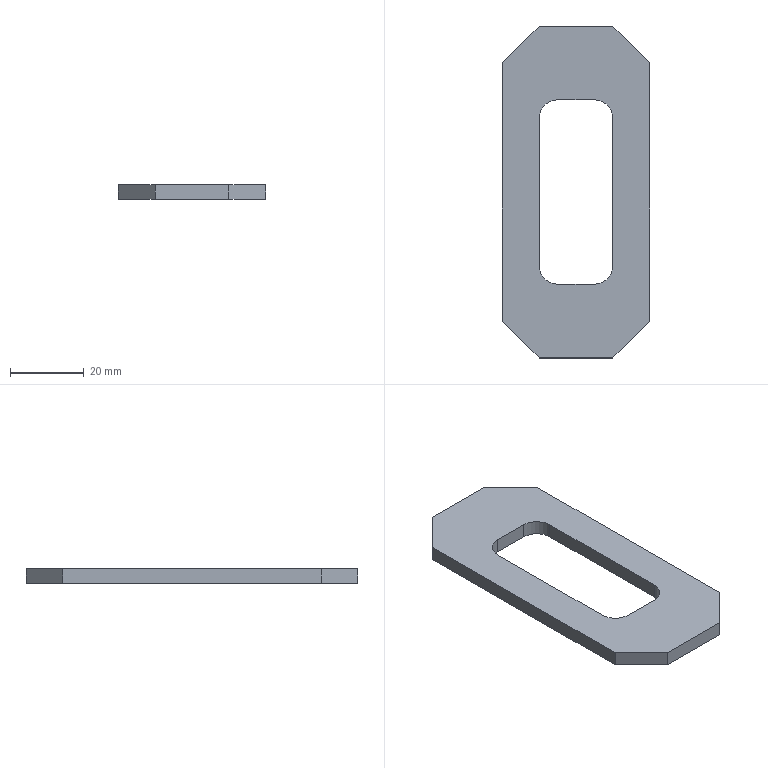Component | SolidWorks | THK-A1029RectangularTubeInnerSealingPlate-2 | 1 solid | 18 faces | box 40 x 90 x 4 mm | volume 9686 mm3 | plane 14 | cylinder 4 | commonest cylinder face diameters 10 x4 | material Q235A
build123d program:
from build123d import *

# Parameters (mm, degrees)
SKETCH1_W           = 40
SKETCH1_H           = 90
BOSS_EXTRUDE1_DEPTH = 2
CUT_EXTRUDE1_DEPTH  = 50.406
CHAMFER1_SIZE       = 10


with BuildPart() as part:
    # Sketch1 → Boss-Extrude1 (new, symmetric)
    with BuildSketch(Plane.XY):
        Rectangle(SKETCH1_W, SKETCH1_H)
    extrude(amount=BOSS_EXTRUDE1_DEPTH, both=True)

    # Sketch2 → Cut-Extrude1 (cut, through all)
    with BuildSketch(Plane.XY.offset(2)):
        with BuildLine():
            Line((-5, -25), (5, -25))
            ThreePointArc((5, -25), (8.536, -23.536), (10, -20))
            Line((10, -20), (10, 20))
            ThreePointArc((10, 20), (8.536, 23.536), (5, 25))
            Line((5, 25), (-5, 25))
            ThreePointArc((-5, 25), (-8.536, 23.536), (-10, 20))
            Line((-10, 20), (-10, -20))
            ThreePointArc((-10, -20), (-8.536, -23.536), (-5, -25))
        make_face()
    extrude(amount=-CUT_EXTRUDE1_DEPTH, mode=Mode.SUBTRACT)

    # Chamfer1
    chamfer1_edges = [part.edges().sort_by_distance(p)[0] for p in [
        (20, -45, 0),
        (-20, -45, 0),
        (-20, 45, 0),
        (20, 45, 0),
    ]]
    chamfer(chamfer1_edges, length=CHAMFER1_SIZE)


solid = part.part

# Placed as in the assembly
solid = solid.moved(Location((-155, -105, -293), (0, 0, 0)))
STEP:
#1=CARTESIAN_POINT('',(-5.315,-5.512,-11.457));
#2=VERTEX_POINT('',#1);
#3=CARTESIAN_POINT('',(-5.315,-2.756,-11.457));
#4=VERTEX_POINT('',#3);
#5=CARTESIAN_POINT('',(-5.315,-5.906,-11.457));
#6=DIRECTION('',(0.,1.,0.));
#7=VECTOR('',#6,39.37);
#8=LINE('',#5,#7);
#9=EDGE_CURVE('',#2,#4,#8,.T.);
#10=ORIENTED_EDGE('',*,*,#9,.F.);
#11=CARTESIAN_POINT('',(-5.315,-5.512,-11.614));
#12=VERTEX_POINT('',#11);
#13=CARTESIAN_POINT('',(-5.315,-5.512,-11.457));
#14=DIRECTION('',(0.,0.,-1.));
#15=VECTOR('',#14,39.37);
#16=LINE('',#13,#15);
#17=EDGE_CURVE('',#2,#12,#16,.T.);
#18=ORIENTED_EDGE('',*,*,#17,.T.);
#19=CARTESIAN_POINT('',(-5.315,-2.756,-11.614));
#20=VERTEX_POINT('',#19);
#21=CARTESIAN_POINT('',(-5.315,-5.906,-11.614));
#22=DIRECTION('',(0.,1.,0.));
#23=VECTOR('',#22,39.37);
#24=LINE('',#21,#23);
#25=EDGE_CURVE('',#12,#20,#24,.T.);
#26=ORIENTED_EDGE('',*,*,#25,.T.);
#27=CARTESIAN_POINT('',(-5.315,-2.756,-11.457));
#28=DIRECTION('',(0.,0.,1.));
#29=VECTOR('',#28,39.37);
#30=LINE('',#27,#29);
#31=EDGE_CURVE('',#20,#4,#30,.T.);
#32=ORIENTED_EDGE('',*,*,#31,.T.);
#33=EDGE_LOOP('',(#10,#18,#26,#32));
#34=FACE_OUTER_BOUND('',#33,.T.);
#35=CARTESIAN_POINT('',(-5.315,-5.906,-11.457));
#36=DIRECTION('',(-1.,0.,0.));
#37=DIRECTION('',(0.,0.,1.));
#38=AXIS2_PLACEMENT_3D('',#35,#36,#37);
#39=PLANE('',#38);
#40=ADVANCED_FACE('',(#34),#39,.F.);
#41=CARTESIAN_POINT('',(-5.709,-2.362,-11.614));
#42=VERTEX_POINT('',#41);
#43=CARTESIAN_POINT('',(-6.496,-2.362,-11.614));
#44=VERTEX_POINT('',#43);
#45=CARTESIAN_POINT('',(-6.89,-2.362,-11.614));
#46=DIRECTION('',(-1.,0.,0.));
#47=VECTOR('',#46,39.37);
#48=LINE('',#45,#47);
#49=EDGE_CURVE('',#42,#44,#48,.T.);
#50=ORIENTED_EDGE('',*,*,#49,.T.);
#51=CARTESIAN_POINT('',(-6.496,-2.362,-11.457));
#52=VERTEX_POINT('',#51);
#53=CARTESIAN_POINT('',(-6.496,-2.362,-11.457));
#54=DIRECTION('',(0.,0.,1.));
#55=VECTOR('',#54,39.37);
#56=LINE('',#53,#55);
#57=EDGE_CURVE('',#44,#52,#56,.T.);
#58=ORIENTED_EDGE('',*,*,#57,.T.);
#59=CARTESIAN_POINT('',(-5.709,-2.362,-11.457));
#60=VERTEX_POINT('',#59);
#61=CARTESIAN_POINT('',(-6.89,-2.362,-11.457));
#62=DIRECTION('',(-1.,0.,0.));
#63=VECTOR('',#62,39.37);
#64=LINE('',#61,#63);
#65=EDGE_CURVE('',#60,#52,#64,.T.);
#66=ORIENTED_EDGE('',*,*,#65,.F.);
#67=CARTESIAN_POINT('',(-5.709,-2.362,-11.457));
#68=DIRECTION('',(0.,0.,-1.));
#69=VECTOR('',#68,39.37);
#70=LINE('',#67,#69);
#71=EDGE_CURVE('',#60,#42,#70,.T.);
#72=ORIENTED_EDGE('',*,*,#71,.T.);
#73=EDGE_LOOP('',(#50,#58,#66,#72));
#74=FACE_OUTER_BOUND('',#73,.T.);
#75=CARTESIAN_POINT('',(-6.89,-2.362,-11.457));
#76=DIRECTION('',(0.,-1.,0.));
#77=DIRECTION('',(0.,0.,-1.));
#78=AXIS2_PLACEMENT_3D('',#75,#76,#77);
#79=PLANE('',#78);
#80=ADVANCED_FACE('',(#74),#79,.F.);
#81=CARTESIAN_POINT('',(-6.89,-2.756,-11.614));
#82=VERTEX_POINT('',#81);
#83=CARTESIAN_POINT('',(-6.89,-5.512,-11.614));
#84=VERTEX_POINT('',#83);
#85=CARTESIAN_POINT('',(-6.89,-5.906,-11.614));
#86=DIRECTION('',(0.,-1.,0.));
#87=VECTOR('',#86,39.37);
#88=LINE('',#85,#87);
#89=EDGE_CURVE('',#82,#84,#88,.T.);
#90=ORIENTED_EDGE('',*,*,#89,.T.);
#91=CARTESIAN_POINT('',(-6.89,-5.512,-11.457));
#92=VERTEX_POINT('',#91);
#93=CARTESIAN_POINT('',(-6.89,-5.512,-11.457));
#94=DIRECTION('',(0.,0.,1.));
#95=VECTOR('',#94,39.37);
#96=LINE('',#93,#95);
#97=EDGE_CURVE('',#84,#92,#96,.T.);
#98=ORIENTED_EDGE('',*,*,#97,.T.);
#99=CARTESIAN_POINT('',(-6.89,-2.756,-11.457));
#100=VERTEX_POINT('',#99);
#101=CARTESIAN_POINT('',(-6.89,-5.906,-11.457));
#102=DIRECTION('',(0.,-1.,0.));
#103=VECTOR('',#102,39.37);
#104=LINE('',#101,#103);
#105=EDGE_CURVE('',#100,#92,#104,.T.);
#106=ORIENTED_EDGE('',*,*,#105,.F.);
#107=CARTESIAN_POINT('',(-6.89,-2.756,-11.457));
#108=DIRECTION('',(0.,0.,-1.));
#109=VECTOR('',#108,39.37);
#110=LINE('',#107,#109);
#111=EDGE_CURVE('',#100,#82,#110,.T.);
#112=ORIENTED_EDGE('',*,*,#111,.T.);
#113=EDGE_LOOP('',(#90,#98,#106,#112));
#114=FACE_OUTER_BOUND('',#113,.T.);
#115=CARTESIAN_POINT('',(-6.89,-5.906,-11.457));
#116=DIRECTION('',(1.,0.,0.));
#117=DIRECTION('',(0.,0.,-1.));
#118=AXIS2_PLACEMENT_3D('',#115,#116,#117);
#119=PLANE('',#118);
#120=ADVANCED_FACE('',(#114),#119,.F.);
#121=CARTESIAN_POINT('',(-6.496,-5.906,-11.614));
#122=VERTEX_POINT('',#121);
#123=CARTESIAN_POINT('',(-5.709,-5.906,-11.614));
#124=VERTEX_POINT('',#123);
#125=CARTESIAN_POINT('',(-6.89,-5.906,-11.614));
#126=DIRECTION('',(1.,0.,0.));
#127=VECTOR('',#126,39.37);
#128=LINE('',#125,#127);
#129=EDGE_CURVE('',#122,#124,#128,.T.);
#130=ORIENTED_EDGE('',*,*,#129,.T.);
#131=CARTESIAN_POINT('',(-5.709,-5.906,-11.457));
#132=VERTEX_POINT('',#131);
#133=CARTESIAN_POINT('',(-5.709,-5.906,-11.457));
#134=DIRECTION('',(0.,0.,1.));
#135=VECTOR('',#134,39.37);
#136=LINE('',#133,#135);
#137=EDGE_CURVE('',#124,#132,#136,.T.);
#138=ORIENTED_EDGE('',*,*,#137,.T.);
#139=CARTESIAN_POINT('',(-6.496,-5.906,-11.457));
#140=VERTEX_POINT('',#139);
#141=CARTESIAN_POINT('',(-6.89,-5.906,-11.457));
#142=DIRECTION('',(1.,0.,0.));
#143=VECTOR('',#142,39.37);
#144=LINE('',#141,#143);
#145=EDGE_CURVE('',#140,#132,#144,.T.);
#146=ORIENTED_EDGE('',*,*,#145,.F.);
#147=CARTESIAN_POINT('',(-6.496,-5.906,-11.457));
#148=DIRECTION('',(0.,0.,-1.));
#149=VECTOR('',#148,39.37);
#150=LINE('',#147,#149);
#151=EDGE_CURVE('',#140,#122,#150,.T.);
#152=ORIENTED_EDGE('',*,*,#151,.T.);
#153=EDGE_LOOP('',(#130,#138,#146,#152));
#154=FACE_OUTER_BOUND('',#153,.T.);
#155=CARTESIAN_POINT('',(-6.89,-5.906,-11.457));
#156=DIRECTION('',(0.,1.,0.));
#157=DIRECTION('',(0.,0.,1.));
#158=AXIS2_PLACEMENT_3D('',#155,#156,#157);
#159=PLANE('',#158);
#160=ADVANCED_FACE('',(#154),#159,.F.);
#161=CARTESIAN_POINT('',(-6.299,-5.118,-11.457));
#162=VERTEX_POINT('',#161);
#163=CARTESIAN_POINT('',(-5.906,-5.118,-11.457));
#164=VERTEX_POINT('',#163);
#165=CARTESIAN_POINT('',(-6.299,-5.118,-11.457));
#166=DIRECTION('',(1.,0.,0.));
#167=VECTOR('',#166,39.37);
#168=LINE('',#165,#167);
#169=EDGE_CURVE('',#162,#164,#168,.T.);
#170=ORIENTED_EDGE('',*,*,#169,.F.);
#171=CARTESIAN_POINT('',(-6.496,-4.921,-11.457));
#172=VERTEX_POINT('',#171);
#173=CARTESIAN_POINT('',(-6.299,-4.921,-11.457));
#174=DIRECTION('',(0.,0.,1.));
#175=DIRECTION('',(1.,0.,0.));
#176=AXIS2_PLACEMENT_3D('',#173,#174,#175);
#177=CIRCLE('',#176,0.1969);
#178=EDGE_CURVE('',#172,#162,#177,.T.);
#179=ORIENTED_EDGE('',*,*,#178,.F.);
#180=CARTESIAN_POINT('',(-6.496,-3.346,-11.457));
#181=VERTEX_POINT('',#180);
#182=CARTESIAN_POINT('',(-6.496,-4.921,-11.457));
#183=DIRECTION('',(0.,-1.,0.));
#184=VECTOR('',#183,39.37);
#185=LINE('',#182,#184);
#186=EDGE_CURVE('',#181,#172,#185,.T.);
#187=ORIENTED_EDGE('',*,*,#186,.F.);
#188=CARTESIAN_POINT('',(-6.299,-3.15,-11.457));
#189=VERTEX_POINT('',#188);
#190=CARTESIAN_POINT('',(-6.299,-3.346,-11.457));
#191=DIRECTION('',(0.,0.,1.));
#192=DIRECTION('',(-1.,0.,0.));
#193=AXIS2_PLACEMENT_3D('',#190,#191,#192);
#194=CIRCLE('',#193,0.1969);
#195=EDGE_CURVE('',#189,#181,#194,.T.);
#196=ORIENTED_EDGE('',*,*,#195,.F.);
#197=CARTESIAN_POINT('',(-5.906,-3.15,-11.457));
#198=VERTEX_POINT('',#197);
#199=CARTESIAN_POINT('',(-6.299,-3.15,-11.457));
#200=DIRECTION('',(-1.,0.,0.));
#201=VECTOR('',#200,39.37);
#202=LINE('',#199,#201);
#203=EDGE_CURVE('',#198,#189,#202,.T.);
#204=ORIENTED_EDGE('',*,*,#203,.F.);
#205=CARTESIAN_POINT('',(-5.709,-3.346,-11.457));
#206=VERTEX_POINT('',#205);
#207=CARTESIAN_POINT('',(-5.906,-3.346,-11.457));
#208=DIRECTION('',(0.,0.,1.));
#209=DIRECTION('',(-1.,0.,0.));
#210=AXIS2_PLACEMENT_3D('',#207,#208,#209);
#211=CIRCLE('',#210,0.1969);
#212=EDGE_CURVE('',#206,#198,#211,.T.);
#213=ORIENTED_EDGE('',*,*,#212,.F.);
#214=CARTESIAN_POINT('',(-5.709,-4.921,-11.457));
#215=VERTEX_POINT('',#214);
#216=CARTESIAN_POINT('',(-5.709,-4.921,-11.457));
#217=DIRECTION('',(0.,1.,0.));
#218=VECTOR('',#217,39.37);
#219=LINE('',#216,#218);
#220=EDGE_CURVE('',#215,#206,#219,.T.);
#221=ORIENTED_EDGE('',*,*,#220,.F.);
#222=CARTESIAN_POINT('',(-5.906,-4.921,-11.457));
#223=DIRECTION('',(0.,0.,1.));
#224=DIRECTION('',(1.,0.,0.));
#225=AXIS2_PLACEMENT_3D('',#222,#223,#224);
#226=CIRCLE('',#225,0.1969);
#227=EDGE_CURVE('',#164,#215,#226,.T.);
#228=ORIENTED_EDGE('',*,*,#227,.F.);
#229=EDGE_LOOP('',(#170,#179,#187,#196,#204,#213,#221,#228));
#230=FACE_BOUND('',#229,.T.);
#231=ORIENTED_EDGE('',*,*,#145,.T.);
#232=CARTESIAN_POINT('',(-5.315,-5.512,-11.457));
#233=DIRECTION('',(0.7071,0.7071,0.));
#234=VECTOR('',#233,39.37);
#235=LINE('',#232,#234);
#236=EDGE_CURVE('',#132,#2,#235,.T.);
#237=ORIENTED_EDGE('',*,*,#236,.T.);
#238=ORIENTED_EDGE('',*,*,#9,.T.);
#239=CARTESIAN_POINT('',(-5.709,-2.362,-11.457));
#240=DIRECTION('',(-0.7071,0.7071,0.));
#241=VECTOR('',#240,39.37);
#242=LINE('',#239,#241);
#243=EDGE_CURVE('',#4,#60,#242,.T.);
#244=ORIENTED_EDGE('',*,*,#243,.T.);
#245=ORIENTED_EDGE('',*,*,#65,.T.);
#246=CARTESIAN_POINT('',(-6.89,-2.756,-11.457));
#247=DIRECTION('',(-0.7071,-0.7071,0.));
#248=VECTOR('',#247,39.37);
#249=LINE('',#246,#248);
#250=EDGE_CURVE('',#52,#100,#249,.T.);
#251=ORIENTED_EDGE('',*,*,#250,.T.);
#252=ORIENTED_EDGE('',*,*,#105,.T.);
#253=CARTESIAN_POINT('',(-6.496,-5.906,-11.457));
#254=DIRECTION('',(0.7071,-0.7071,0.));
#255=VECTOR('',#254,39.37);
#256=LINE('',#253,#255);
#257=EDGE_CURVE('',#92,#140,#256,.T.);
#258=ORIENTED_EDGE('',*,*,#257,.T.);
#259=EDGE_LOOP('',(#231,#237,#238,#244,#245,#251,#252,#258));
#260=FACE_OUTER_BOUND('',#259,.T.);
#261=CARTESIAN_POINT('',(-6.102,-4.134,-11.457));
#262=DIRECTION('',(0.,0.,-1.));
#263=DIRECTION('',(-1.,0.,0.));
#264=AXIS2_PLACEMENT_3D('',#261,#262,#263);
#265=PLANE('',#264);
#266=ADVANCED_FACE('',(#230,#260),#265,.F.);
#267=CARTESIAN_POINT('',(-6.496,-4.921,-11.614));
#268=VERTEX_POINT('',#267);
#269=CARTESIAN_POINT('',(-6.299,-5.118,-11.614));
#270=VERTEX_POINT('',#269);
#271=CARTESIAN_POINT('',(-6.299,-4.921,-11.614));
#272=DIRECTION('',(0.,0.,1.));
#273=DIRECTION('',(1.,0.,0.));
#274=AXIS2_PLACEMENT_3D('',#271,#272,#273);
#275=CIRCLE('',#274,0.1969);
#276=EDGE_CURVE('',#268,#270,#275,.T.);
#277=ORIENTED_EDGE('',*,*,#276,.T.);
#278=CARTESIAN_POINT('',(-5.906,-5.118,-11.614));
#279=VERTEX_POINT('',#278);
#280=CARTESIAN_POINT('',(-6.299,-5.118,-11.614));
#281=DIRECTION('',(1.,0.,0.));
#282=VECTOR('',#281,39.37);
#283=LINE('',#280,#282);
#284=EDGE_CURVE('',#270,#279,#283,.T.);
#285=ORIENTED_EDGE('',*,*,#284,.T.);
#286=CARTESIAN_POINT('',(-5.709,-4.921,-11.614));
#287=VERTEX_POINT('',#286);
#288=CARTESIAN_POINT('',(-5.906,-4.921,-11.614));
#289=DIRECTION('',(0.,0.,1.));
#290=DIRECTION('',(1.,0.,0.));
#291=AXIS2_PLACEMENT_3D('',#288,#289,#290);
#292=CIRCLE('',#291,0.1969);
#293=EDGE_CURVE('',#279,#287,#292,.T.);
#294=ORIENTED_EDGE('',*,*,#293,.T.);
#295=CARTESIAN_POINT('',(-5.709,-3.346,-11.614));
#296=VERTEX_POINT('',#295);
#297=CARTESIAN_POINT('',(-5.709,-4.921,-11.614));
#298=DIRECTION('',(0.,1.,0.));
#299=VECTOR('',#298,39.37);
#300=LINE('',#297,#299);
#301=EDGE_CURVE('',#287,#296,#300,.T.);
#302=ORIENTED_EDGE('',*,*,#301,.T.);
#303=CARTESIAN_POINT('',(-5.906,-3.15,-11.614));
#304=VERTEX_POINT('',#303);
#305=CARTESIAN_POINT('',(-5.906,-3.346,-11.614));
#306=DIRECTION('',(0.,0.,1.));
#307=DIRECTION('',(-1.,0.,0.));
#308=AXIS2_PLACEMENT_3D('',#305,#306,#307);
#309=CIRCLE('',#308,0.1969);
#310=EDGE_CURVE('',#296,#304,#309,.T.);
#311=ORIENTED_EDGE('',*,*,#310,.T.);
#312=CARTESIAN_POINT('',(-6.299,-3.15,-11.614));
#313=VERTEX_POINT('',#312);
#314=CARTESIAN_POINT('',(-6.299,-3.15,-11.614));
#315=DIRECTION('',(-1.,0.,0.));
#316=VECTOR('',#315,39.37);
#317=LINE('',#314,#316);
#318=EDGE_CURVE('',#304,#313,#317,.T.);
#319=ORIENTED_EDGE('',*,*,#318,.T.);
#320=CARTESIAN_POINT('',(-6.496,-3.346,-11.614));
#321=VERTEX_POINT('',#320);
#322=CARTESIAN_POINT('',(-6.299,-3.346,-11.614));
#323=DIRECTION('',(0.,0.,1.));
#324=DIRECTION('',(-1.,0.,0.));
#325=AXIS2_PLACEMENT_3D('',#322,#323,#324);
#326=CIRCLE('',#325,0.1969);
#327=EDGE_CURVE('',#313,#321,#326,.T.);
#328=ORIENTED_EDGE('',*,*,#327,.T.);
#329=CARTESIAN_POINT('',(-6.496,-4.921,-11.614));
#330=DIRECTION('',(0.,-1.,0.));
#331=VECTOR('',#330,39.37);
#332=LINE('',#329,#331);
#333=EDGE_CURVE('',#321,#268,#332,.T.);
#334=ORIENTED_EDGE('',*,*,#333,.T.);
#335=EDGE_LOOP('',(#277,#285,#294,#302,#311,#319,#328,#334));
#336=FACE_BOUND('',#335,.T.);
#337=ORIENTED_EDGE('',*,*,#25,.F.);
#338=CARTESIAN_POINT('',(-5.02,-5.217,-11.614));
#339=DIRECTION('',(-0.7071,-0.7071,0.));
#340=VECTOR('',#339,39.37);
#341=LINE('',#338,#340);
#342=EDGE_CURVE('',#12,#124,#341,.T.);
#343=ORIENTED_EDGE('',*,*,#342,.T.);
#344=ORIENTED_EDGE('',*,*,#129,.F.);
#345=CARTESIAN_POINT('',(-7.185,-5.217,-11.614));
#346=DIRECTION('',(-0.7071,0.7071,0.));
#347=VECTOR('',#346,39.37);
#348=LINE('',#345,#347);
#349=EDGE_CURVE('',#122,#84,#348,.T.);
#350=ORIENTED_EDGE('',*,*,#349,.T.);
#351=ORIENTED_EDGE('',*,*,#89,.F.);
#352=CARTESIAN_POINT('',(-7.185,-3.051,-11.614));
#353=DIRECTION('',(0.7071,0.7071,0.));
#354=VECTOR('',#353,39.37);
#355=LINE('',#352,#354);
#356=EDGE_CURVE('',#82,#44,#355,.T.);
#357=ORIENTED_EDGE('',*,*,#356,.T.);
#358=ORIENTED_EDGE('',*,*,#49,.F.);
#359=CARTESIAN_POINT('',(-5.02,-3.051,-11.614));
#360=DIRECTION('',(0.7071,-0.7071,0.));
#361=VECTOR('',#360,39.37);
#362=LINE('',#359,#361);
#363=EDGE_CURVE('',#42,#20,#362,.T.);
#364=ORIENTED_EDGE('',*,*,#363,.T.);
#365=EDGE_LOOP('',(#337,#343,#344,#350,#351,#357,#358,#364));
#366=FACE_OUTER_BOUND('',#365,.T.);
#367=CARTESIAN_POINT('',(-6.102,-4.134,-11.614));
#368=DIRECTION('',(0.,0.,-1.));
#369=DIRECTION('',(-1.,0.,0.));
#370=AXIS2_PLACEMENT_3D('',#367,#368,#369);
#371=PLANE('',#370);
#372=ADVANCED_FACE('',(#336,#366),#371,.T.);
#373=ORIENTED_EDGE('',*,*,#178,.T.);
#374=CARTESIAN_POINT('',(-6.299,-5.118,-11.614));
#375=DIRECTION('',(0.,0.,1.));
#376=VECTOR('',#375,39.37);
#377=LINE('',#374,#376);
#378=EDGE_CURVE('',#270,#162,#377,.T.);
#379=ORIENTED_EDGE('',*,*,#378,.F.);
#380=ORIENTED_EDGE('',*,*,#276,.F.);
#381=CARTESIAN_POINT('',(-6.496,-4.921,-11.614));
#382=DIRECTION('',(0.,0.,1.));
#383=VECTOR('',#382,39.37);
#384=LINE('',#381,#383);
#385=EDGE_CURVE('',#268,#172,#384,.T.);
#386=ORIENTED_EDGE('',*,*,#385,.T.);
#387=EDGE_LOOP('',(#373,#379,#380,#386));
#388=FACE_OUTER_BOUND('',#387,.T.);
#389=CARTESIAN_POINT('',(-6.299,-4.921,-11.614));
#390=DIRECTION('',(0.,0.,1.));
#391=DIRECTION('',(1.,0.,0.));
#392=AXIS2_PLACEMENT_3D('',#389,#390,#391);
#393=CYLINDRICAL_SURFACE('',#392,0.1969);
#394=ADVANCED_FACE('',(#388),#393,.F.);
#395=ORIENTED_EDGE('',*,*,#186,.T.);
#396=ORIENTED_EDGE('',*,*,#385,.F.);
#397=ORIENTED_EDGE('',*,*,#333,.F.);
#398=CARTESIAN_POINT('',(-6.496,-3.346,-11.614));
#399=DIRECTION('',(0.,0.,1.));
#400=VECTOR('',#399,39.37);
#401=LINE('',#398,#400);
#402=EDGE_CURVE('',#321,#181,#401,.T.);
#403=ORIENTED_EDGE('',*,*,#402,.T.);
#404=EDGE_LOOP('',(#395,#396,#397,#403));
#405=FACE_OUTER_BOUND('',#404,.T.);
#406=CARTESIAN_POINT('',(-6.496,-4.921,-11.614));
#407=DIRECTION('',(-1.,0.,0.));
#408=DIRECTION('',(0.,0.,1.));
#409=AXIS2_PLACEMENT_3D('',#406,#407,#408);
#410=PLANE('',#409);
#411=ADVANCED_FACE('',(#405),#410,.F.);
#412=ORIENTED_EDGE('',*,*,#195,.T.);
#413=ORIENTED_EDGE('',*,*,#402,.F.);
#414=ORIENTED_EDGE('',*,*,#327,.F.);
#415=CARTESIAN_POINT('',(-6.299,-3.15,-11.614));
#416=DIRECTION('',(0.,0.,1.));
#417=VECTOR('',#416,39.37);
#418=LINE('',#415,#417);
#419=EDGE_CURVE('',#313,#189,#418,.T.);
#420=ORIENTED_EDGE('',*,*,#419,.T.);
#421=EDGE_LOOP('',(#412,#413,#414,#420));
#422=FACE_OUTER_BOUND('',#421,.T.);
#423=CARTESIAN_POINT('',(-6.299,-3.346,-11.614));
#424=DIRECTION('',(0.,0.,1.));
#425=DIRECTION('',(1.,0.,0.));
#426=AXIS2_PLACEMENT_3D('',#423,#424,#425);
#427=CYLINDRICAL_SURFACE('',#426,0.1969);
#428=ADVANCED_FACE('',(#422),#427,.F.);
#429=ORIENTED_EDGE('',*,*,#203,.T.);
#430=ORIENTED_EDGE('',*,*,#419,.F.);
#431=ORIENTED_EDGE('',*,*,#318,.F.);
#432=CARTESIAN_POINT('',(-5.906,-3.15,-11.614));
#433=DIRECTION('',(0.,0.,1.));
#434=VECTOR('',#433,39.37);
#435=LINE('',#432,#434);
#436=EDGE_CURVE('',#304,#198,#435,.T.);
#437=ORIENTED_EDGE('',*,*,#436,.T.);
#438=EDGE_LOOP('',(#429,#430,#431,#437));
#439=FACE_OUTER_BOUND('',#438,.T.);
#440=CARTESIAN_POINT('',(-6.299,-3.15,-11.614));
#441=DIRECTION('',(0.,1.,0.));
#442=DIRECTION('',(0.,0.,1.));
#443=AXIS2_PLACEMENT_3D('',#440,#441,#442);
#444=PLANE('',#443);
#445=ADVANCED_FACE('',(#439),#444,.F.);
#446=ORIENTED_EDGE('',*,*,#212,.T.);
#447=ORIENTED_EDGE('',*,*,#436,.F.);
#448=ORIENTED_EDGE('',*,*,#310,.F.);
#449=CARTESIAN_POINT('',(-5.709,-3.346,-11.614));
#450=DIRECTION('',(0.,0.,1.));
#451=VECTOR('',#450,39.37);
#452=LINE('',#449,#451);
#453=EDGE_CURVE('',#296,#206,#452,.T.);
#454=ORIENTED_EDGE('',*,*,#453,.T.);
#455=EDGE_LOOP('',(#446,#447,#448,#454));
#456=FACE_OUTER_BOUND('',#455,.T.);
#457=CARTESIAN_POINT('',(-5.906,-3.346,-11.614));
#458=DIRECTION('',(0.,0.,1.));
#459=DIRECTION('',(1.,0.,0.));
#460=AXIS2_PLACEMENT_3D('',#457,#458,#459);
#461=CYLINDRICAL_SURFACE('',#460,0.1969);
#462=ADVANCED_FACE('',(#456),#461,.F.);
#463=ORIENTED_EDGE('',*,*,#220,.T.);
#464=ORIENTED_EDGE('',*,*,#453,.F.);
#465=ORIENTED_EDGE('',*,*,#301,.F.);
#466=CARTESIAN_POINT('',(-5.709,-4.921,-11.614));
#467=DIRECTION('',(0.,0.,1.));
#468=VECTOR('',#467,39.37);
#469=LINE('',#466,#468);
#470=EDGE_CURVE('',#287,#215,#469,.T.);
#471=ORIENTED_EDGE('',*,*,#470,.T.);
#472=EDGE_LOOP('',(#463,#464,#465,#471));
#473=FACE_OUTER_BOUND('',#472,.T.);
#474=CARTESIAN_POINT('',(-5.709,-4.921,-11.614));
#475=DIRECTION('',(1.,0.,0.));
#476=DIRECTION('',(0.,0.,-1.));
#477=AXIS2_PLACEMENT_3D('',#474,#475,#476);
#478=PLANE('',#477);
#479=ADVANCED_FACE('',(#473),#478,.F.);
#480=ORIENTED_EDGE('',*,*,#227,.T.);
#481=ORIENTED_EDGE('',*,*,#470,.F.);
#482=ORIENTED_EDGE('',*,*,#293,.F.);
#483=CARTESIAN_POINT('',(-5.906,-5.118,-11.614));
#484=DIRECTION('',(0.,0.,1.));
#485=VECTOR('',#484,39.37);
#486=LINE('',#483,#485);
#487=EDGE_CURVE('',#279,#164,#486,.T.);
#488=ORIENTED_EDGE('',*,*,#487,.T.);
#489=EDGE_LOOP('',(#480,#481,#482,#488));
#490=FACE_OUTER_BOUND('',#489,.T.);
#491=CARTESIAN_POINT('',(-5.906,-4.921,-11.614));
#492=DIRECTION('',(0.,0.,1.));
#493=DIRECTION('',(1.,0.,0.));
#494=AXIS2_PLACEMENT_3D('',#491,#492,#493);
#495=CYLINDRICAL_SURFACE('',#494,0.1969);
#496=ADVANCED_FACE('',(#490),#495,.F.);
#497=ORIENTED_EDGE('',*,*,#169,.T.);
#498=ORIENTED_EDGE('',*,*,#487,.F.);
#499=ORIENTED_EDGE('',*,*,#284,.F.);
#500=ORIENTED_EDGE('',*,*,#378,.T.);
#501=EDGE_LOOP('',(#497,#498,#499,#500));
#502=FACE_OUTER_BOUND('',#501,.T.);
#503=CARTESIAN_POINT('',(-6.299,-5.118,-11.614));
#504=DIRECTION('',(0.,-1.,0.));
#505=DIRECTION('',(0.,0.,-1.));
#506=AXIS2_PLACEMENT_3D('',#503,#504,#505);
#507=PLANE('',#506);
#508=ADVANCED_FACE('',(#502),#507,.F.);
#509=ORIENTED_EDGE('',*,*,#236,.F.);
#510=ORIENTED_EDGE('',*,*,#137,.F.);
#511=ORIENTED_EDGE('',*,*,#342,.F.);
#512=ORIENTED_EDGE('',*,*,#17,.F.);
#513=EDGE_LOOP('',(#509,#510,#511,#512));
#514=FACE_OUTER_BOUND('',#513,.T.);
#515=CARTESIAN_POINT('',(-5.315,-5.512,-11.457));
#516=DIRECTION('',(-0.7071,0.7071,0.));
#517=DIRECTION('',(0.,0.,-1.));
#518=AXIS2_PLACEMENT_3D('',#515,#516,#517);
#519=PLANE('',#518);
#520=ADVANCED_FACE('',(#514),#519,.F.);
#521=ORIENTED_EDGE('',*,*,#257,.F.);
#522=ORIENTED_EDGE('',*,*,#97,.F.);
#523=ORIENTED_EDGE('',*,*,#349,.F.);
#524=ORIENTED_EDGE('',*,*,#151,.F.);
#525=EDGE_LOOP('',(#521,#522,#523,#524));
#526=FACE_OUTER_BOUND('',#525,.T.);
#527=CARTESIAN_POINT('',(-6.496,-5.906,-11.457));
#528=DIRECTION('',(0.7071,0.7071,0.));
#529=DIRECTION('',(0.,0.,-1.));
#530=AXIS2_PLACEMENT_3D('',#527,#528,#529);
#531=PLANE('',#530);
#532=ADVANCED_FACE('',(#526),#531,.F.);
#533=ORIENTED_EDGE('',*,*,#250,.F.);
#534=ORIENTED_EDGE('',*,*,#57,.F.);
#535=ORIENTED_EDGE('',*,*,#356,.F.);
#536=ORIENTED_EDGE('',*,*,#111,.F.);
#537=EDGE_LOOP('',(#533,#534,#535,#536));
#538=FACE_OUTER_BOUND('',#537,.T.);
#539=CARTESIAN_POINT('',(-6.89,-2.756,-11.457));
#540=DIRECTION('',(0.7071,-0.7071,0.));
#541=DIRECTION('',(0.,0.,-1.));
#542=AXIS2_PLACEMENT_3D('',#539,#540,#541);
#543=PLANE('',#542);
#544=ADVANCED_FACE('',(#538),#543,.F.);
#545=ORIENTED_EDGE('',*,*,#243,.F.);
#546=ORIENTED_EDGE('',*,*,#31,.F.);
#547=ORIENTED_EDGE('',*,*,#363,.F.);
#548=ORIENTED_EDGE('',*,*,#71,.F.);
#549=EDGE_LOOP('',(#545,#546,#547,#548));
#550=FACE_OUTER_BOUND('',#549,.T.);
#551=CARTESIAN_POINT('',(-5.709,-2.362,-11.457));
#552=DIRECTION('',(-0.7071,-0.7071,0.));
#553=DIRECTION('',(0.,0.,-1.));
#554=AXIS2_PLACEMENT_3D('',#551,#552,#553);
#555=PLANE('',#554);
#556=ADVANCED_FACE('',(#550),#555,.F.);
#557=CLOSED_SHELL('',(#40,#80,#120,#160,#266,#372,#394,#411,#428,#445,#462,#479,#496,#508,#520,#532,#544,#556));
#558=MANIFOLD_SOLID_BREP('',#557);
#559=CARTESIAN_POINT('',(0.,0.,0.));
#560=DIRECTION('',(0.,0.,1.));
#561=DIRECTION('',(1.,0.,0.));
#562=AXIS2_PLACEMENT_3D('',#559,#560,#561);
#563=(LENGTH_UNIT()NAMED_UNIT(*)SI_UNIT($,.METRE.));
#564=LENGTH_MEASURE_WITH_UNIT(LENGTH_MEASURE(0.0254),#563);
#565=DIMENSIONAL_EXPONENTS(1.,0.,0.,0.,0.,0.,0.);
#566=(CONVERSION_BASED_UNIT('',#564)LENGTH_UNIT()NAMED_UNIT(#565));
#567=UNCERTAINTY_MEASURE_WITH_UNIT(LENGTH_MEASURE(0.00001),#566,'','');
#568=(NAMED_UNIT(*)PLANE_ANGLE_UNIT()SI_UNIT($,.RADIAN.));
#569=(NAMED_UNIT(*)SI_UNIT($,.STERADIAN.)SOLID_ANGLE_UNIT());
#570=(GEOMETRIC_REPRESENTATION_CONTEXT(3)GLOBAL_UNCERTAINTY_ASSIGNED_CONTEXT((#567))GLOBAL_UNIT_ASSIGNED_CONTEXT((#566,#568,#569))REPRESENTATION_CONTEXT('',''));
#571=ADVANCED_BREP_SHAPE_REPRESENTATION('',(#558,#562),#570);
#572=COLOUR_RGB('',0.7922,0.8196,0.9333);
#573=FILL_AREA_STYLE_COLOUR('',#572);
#574=FILL_AREA_STYLE('',(#573));
#575=SURFACE_STYLE_FILL_AREA(#574);
#576=SURFACE_SIDE_STYLE('',(#575));
#577=SURFACE_STYLE_USAGE(.BOTH.,#576);
#578=PRESENTATION_STYLE_ASSIGNMENT((#577));
#579=STYLED_ITEM('',(#578),#558);
#580=(LENGTH_UNIT()NAMED_UNIT(*)SI_UNIT($,.METRE.));
#581=LENGTH_MEASURE_WITH_UNIT(LENGTH_MEASURE(0.0254),#580);
#582=DIMENSIONAL_EXPONENTS(1.,0.,0.,0.,0.,0.,0.);
#583=(CONVERSION_BASED_UNIT('',#581)LENGTH_UNIT()NAMED_UNIT(#582));
#584=UNCERTAINTY_MEASURE_WITH_UNIT(LENGTH_MEASURE(0.00001),#583,'','');
#585=(NAMED_UNIT(*)PLANE_ANGLE_UNIT()SI_UNIT($,.RADIAN.));
#586=(NAMED_UNIT(*)SI_UNIT($,.STERADIAN.)SOLID_ANGLE_UNIT());
#587=(GEOMETRIC_REPRESENTATION_CONTEXT(3)GLOBAL_UNCERTAINTY_ASSIGNED_CONTEXT((#584))GLOBAL_UNIT_ASSIGNED_CONTEXT((#583,#585,#586))REPRESENTATION_CONTEXT('',''));
#588=MECHANICAL_DESIGN_GEOMETRIC_PRESENTATION_REPRESENTATION('',(#579),#587);
#589=PRESENTATION_LAYER_ASSIGNMENT('','',(#579));